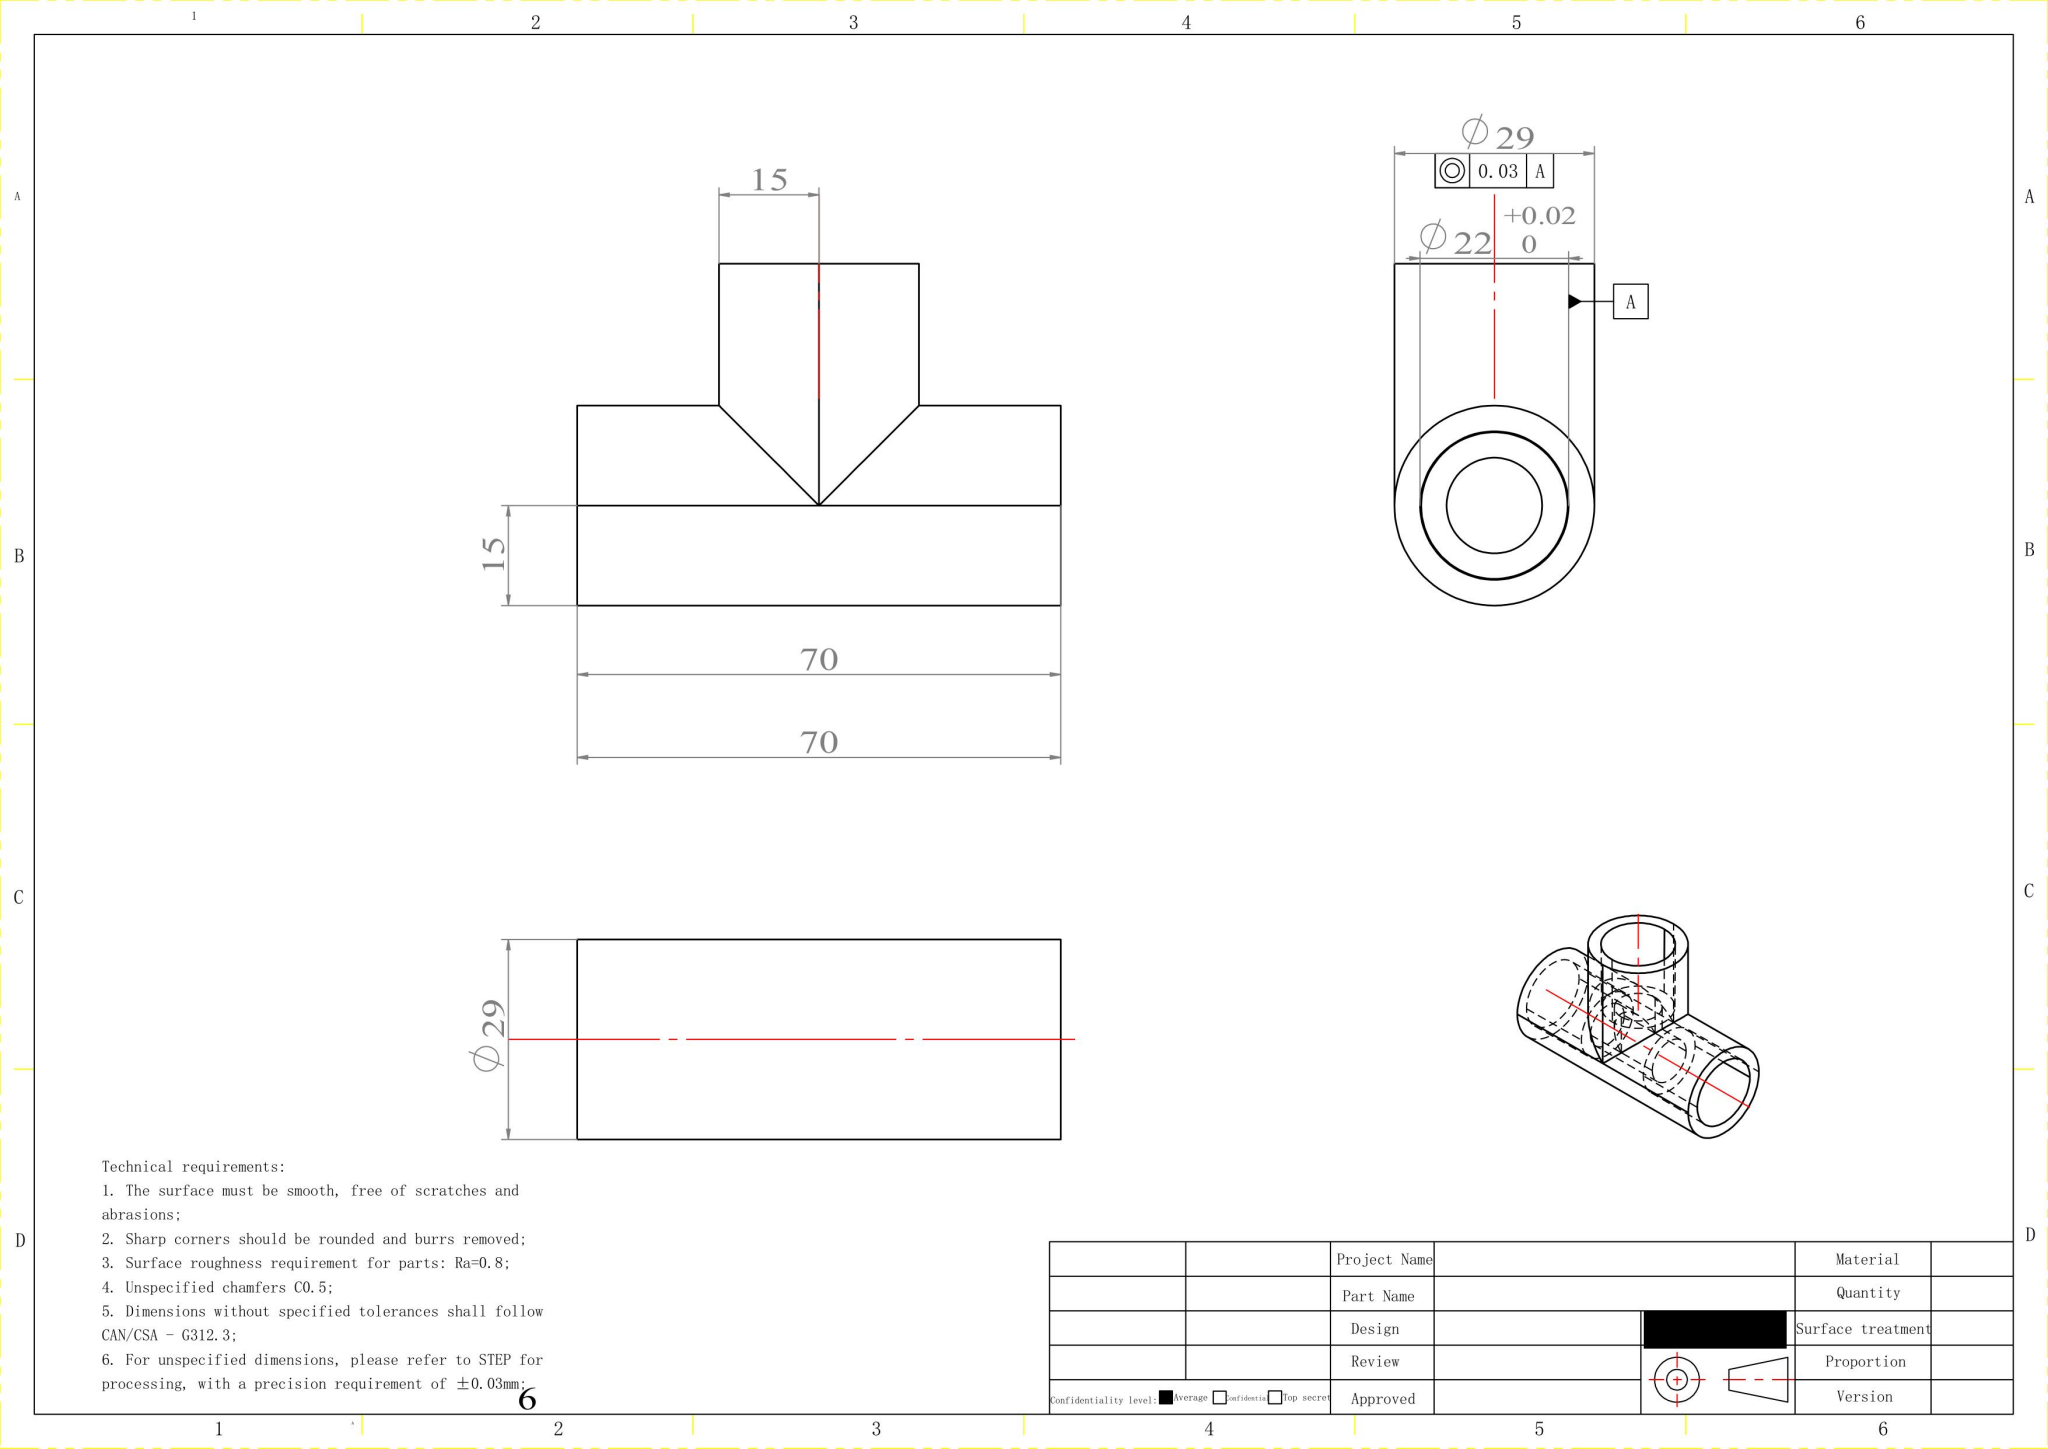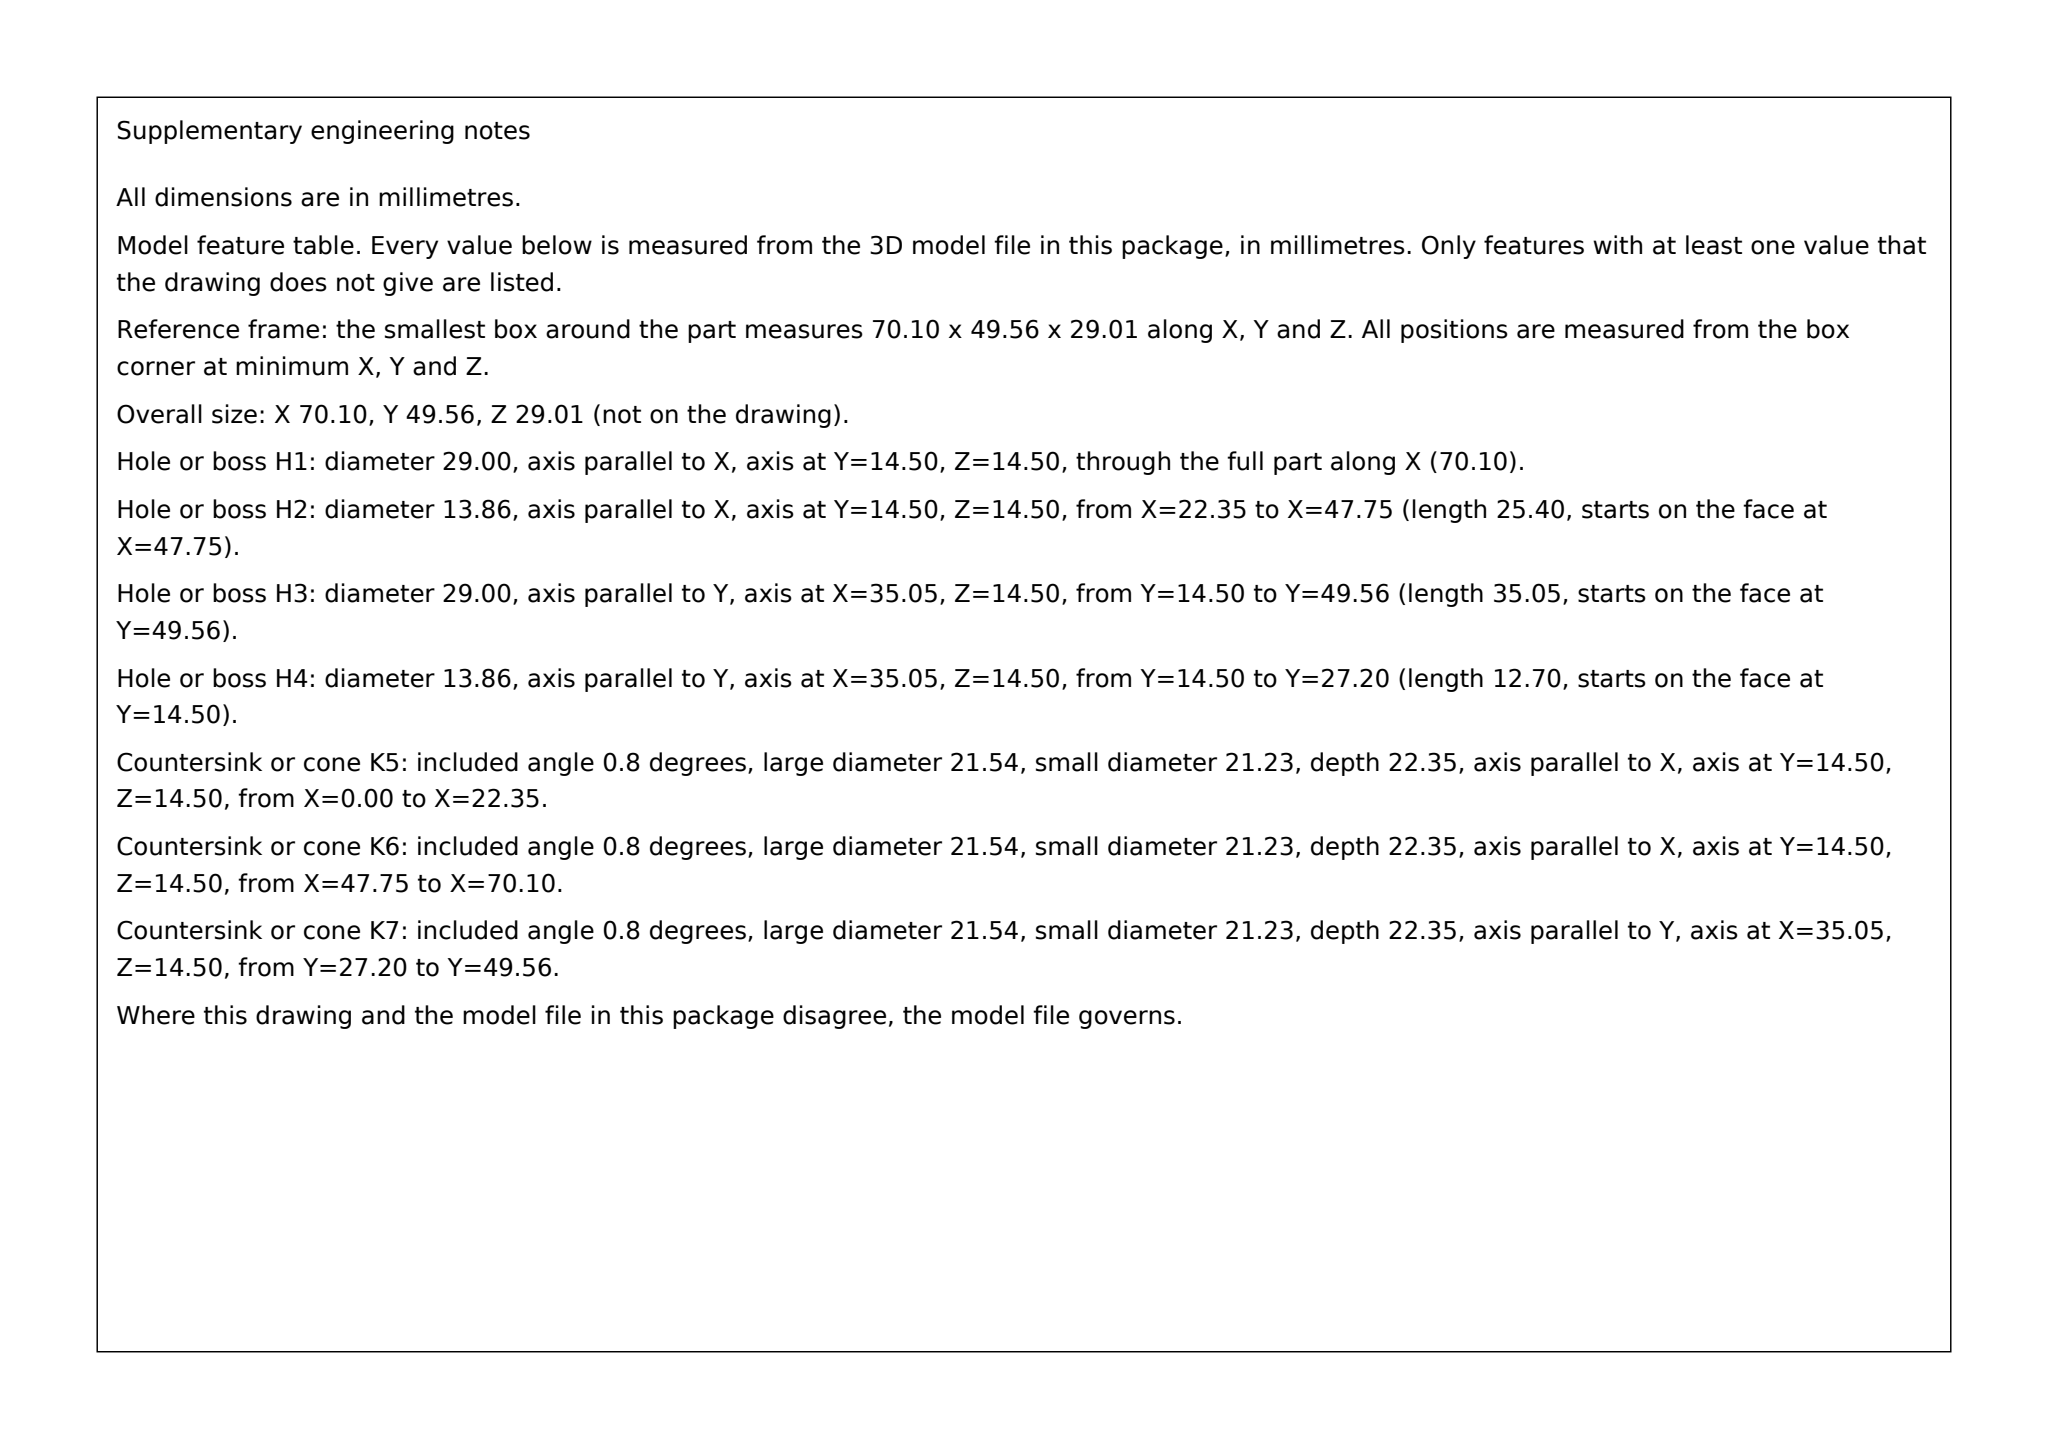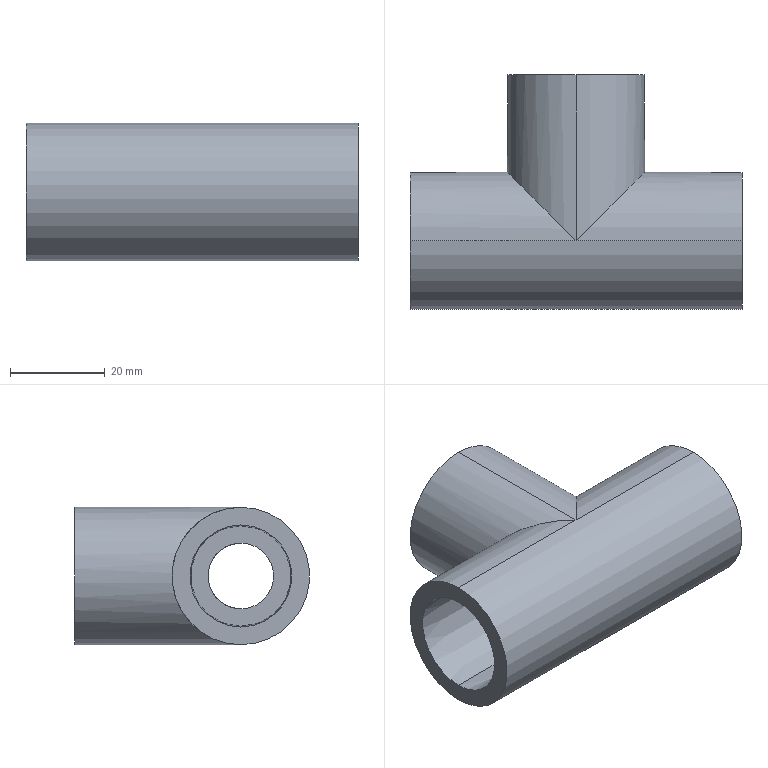Part | SolidWorks | mm | 1 solid | 22 faces | box 70.1 x 49.56 x 29.01 mm | volume 32399 mm3 | cylinder 10 | plane 6 | cone 6 | commonest cylinder face diameters 29.007 x5 13.868 x5
STEP:
#1=CARTESIAN_POINT('',(35.052,-0.,14.503));
#2=VERTEX_POINT('',#1);
#3=CARTESIAN_POINT('',(0.,0.,14.503));
#4=VERTEX_POINT('',#3);
#5=CARTESIAN_POINT('',(35.052,0.,14.503));
#6=DIRECTION('',(-1.,0.,0.));
#7=VECTOR('',#6,1000.);
#8=LINE('',#5,#7);
#9=EDGE_CURVE('',#2,#4,#8,.T.);
#10=ORIENTED_EDGE('',*,*,#9,.F.);
#11=CARTESIAN_POINT('',(35.052,-0.,-14.503));
#12=VERTEX_POINT('',#11);
#13=CARTESIAN_POINT('',(35.052,0.,-0.));
#14=DIRECTION('',(-1.,-0.,-0.));
#15=DIRECTION('',(0.,-0.,1.));
#16=AXIS2_PLACEMENT_3D('',#13,#14,#15);
#17=CIRCLE('',#16,14.503);
#18=EDGE_CURVE('',#2,#12,#17,.T.);
#19=ORIENTED_EDGE('',*,*,#18,.T.);
#20=CARTESIAN_POINT('',(0.,0.,-14.503));
#21=VERTEX_POINT('',#20);
#22=CARTESIAN_POINT('',(0.,0.,-14.503));
#23=DIRECTION('',(1.,-0.,0.));
#24=VECTOR('',#23,1000.);
#25=LINE('',#22,#24);
#26=EDGE_CURVE('',#21,#12,#25,.T.);
#27=ORIENTED_EDGE('',*,*,#26,.F.);
#28=CARTESIAN_POINT('',(0.,0.,14.503));
#29=CARTESIAN_POINT('',(14.503,14.503,14.503));
#30=CARTESIAN_POINT('',(14.503,14.503,0.));
#31=CARTESIAN_POINT('',(14.503,14.503,-14.503));
#32=CARTESIAN_POINT('',(0.,0.,-14.503));
#33=(BOUNDED_CURVE()B_SPLINE_CURVE(2,(#28,#29,#30,#31,#32),.UNSPECIFIED.,.F.,.F.)B_SPLINE_CURVE_WITH_KNOTS((3,2,3),(0.,0.5,1.),.UNSPECIFIED.)CURVE()GEOMETRIC_REPRESENTATION_ITEM()RATIONAL_B_SPLINE_CURVE((1.,0.7071,1.,0.7071,1.))REPRESENTATION_ITEM(''));
#34=EDGE_CURVE('',#4,#21,#33,.T.);
#35=ORIENTED_EDGE('',*,*,#34,.F.);
#36=EDGE_LOOP('',(#10,#19,#27,#35));
#37=FACE_OUTER_BOUND('',#36,.T.);
#38=CARTESIAN_POINT('',(35.052,0.,-0.));
#39=DIRECTION('',(-1.,0.,-0.));
#40=DIRECTION('',(-0.,0.,1.));
#41=AXIS2_PLACEMENT_3D('',#38,#39,#40);
#42=CYLINDRICAL_SURFACE('',#41,14.503);
#43=ADVANCED_FACE('',(#37),#42,.T.);
#44=CARTESIAN_POINT('',(-35.052,-0.,-14.503));
#45=VERTEX_POINT('',#44);
#46=CARTESIAN_POINT('',(-35.052,-0.,14.503));
#47=VERTEX_POINT('',#46);
#48=CARTESIAN_POINT('',(-35.052,-0.,-0.));
#49=DIRECTION('',(1.,0.,0.));
#50=DIRECTION('',(0.,0.,-1.));
#51=AXIS2_PLACEMENT_3D('',#48,#49,#50);
#52=CIRCLE('',#51,14.503);
#53=EDGE_CURVE('',#45,#47,#52,.T.);
#54=ORIENTED_EDGE('',*,*,#53,.T.);
#55=CARTESIAN_POINT('',(-35.052,0.,14.503));
#56=DIRECTION('',(1.,0.,0.));
#57=VECTOR('',#56,1000.);
#58=LINE('',#55,#57);
#59=EDGE_CURVE('',#47,#4,#58,.T.);
#60=ORIENTED_EDGE('',*,*,#59,.T.);
#61=CARTESIAN_POINT('',(0.,0.,-14.503));
#62=CARTESIAN_POINT('',(-14.503,14.503,-14.503));
#63=CARTESIAN_POINT('',(-14.503,14.503,-0.));
#64=CARTESIAN_POINT('',(-14.503,14.503,14.503));
#65=CARTESIAN_POINT('',(0.,0.,14.503));
#66=(BOUNDED_CURVE()B_SPLINE_CURVE(2,(#61,#62,#63,#64,#65),.UNSPECIFIED.,.F.,.F.)B_SPLINE_CURVE_WITH_KNOTS((3,2,3),(0.,0.5,1.),.UNSPECIFIED.)CURVE()GEOMETRIC_REPRESENTATION_ITEM()RATIONAL_B_SPLINE_CURVE((1.,0.7071,1.,0.7071,1.))REPRESENTATION_ITEM(''));
#67=EDGE_CURVE('',#21,#4,#66,.T.);
#68=ORIENTED_EDGE('',*,*,#67,.F.);
#69=CARTESIAN_POINT('',(-35.052,-0.,-14.503));
#70=DIRECTION('',(1.,0.,0.));
#71=VECTOR('',#70,1000.);
#72=LINE('',#69,#71);
#73=EDGE_CURVE('',#45,#21,#72,.T.);
#74=ORIENTED_EDGE('',*,*,#73,.F.);
#75=EDGE_LOOP('',(#54,#60,#68,#74));
#76=FACE_OUTER_BOUND('',#75,.T.);
#77=CARTESIAN_POINT('',(35.052,0.,-0.));
#78=DIRECTION('',(-1.,0.,-0.));
#79=DIRECTION('',(-0.,0.,1.));
#80=AXIS2_PLACEMENT_3D('',#77,#78,#79);
#81=CYLINDRICAL_SURFACE('',#80,14.503);
#82=ADVANCED_FACE('',(#76),#81,.T.);
#83=CARTESIAN_POINT('',(-12.7,0.,6.934));
#84=VERTEX_POINT('',#83);
#85=CARTESIAN_POINT('',(0.,0.,6.934));
#86=VERTEX_POINT('',#85);
#87=CARTESIAN_POINT('',(-12.7,0.,6.934));
#88=DIRECTION('',(1.,0.,0.));
#89=VECTOR('',#88,1000.);
#90=LINE('',#87,#89);
#91=EDGE_CURVE('',#84,#86,#90,.T.);
#92=ORIENTED_EDGE('',*,*,#91,.F.);
#93=CARTESIAN_POINT('',(-12.7,0.,-6.934));
#94=VERTEX_POINT('',#93);
#95=CARTESIAN_POINT('',(-12.7,0.,0.));
#96=DIRECTION('',(-1.,0.,0.));
#97=DIRECTION('',(0.,-0.,1.));
#98=AXIS2_PLACEMENT_3D('',#95,#96,#97);
#99=CIRCLE('',#98,6.934);
#100=EDGE_CURVE('',#84,#94,#99,.T.);
#101=ORIENTED_EDGE('',*,*,#100,.T.);
#102=CARTESIAN_POINT('',(0.,0.,-6.934));
#103=VERTEX_POINT('',#102);
#104=CARTESIAN_POINT('',(0.,0.,-6.934));
#105=DIRECTION('',(-1.,0.,0.));
#106=VECTOR('',#105,1000.);
#107=LINE('',#104,#106);
#108=EDGE_CURVE('',#103,#94,#107,.T.);
#109=ORIENTED_EDGE('',*,*,#108,.F.);
#110=CARTESIAN_POINT('',(0.,0.,6.934));
#111=CARTESIAN_POINT('',(-13.868,13.868,6.934));
#112=CARTESIAN_POINT('',(-13.868,13.868,-6.934));
#113=CARTESIAN_POINT('',(0.,0.,-6.934));
#114=(BOUNDED_CURVE()B_SPLINE_CURVE(3,(#110,#111,#112,#113),.UNSPECIFIED.,.F.,.F.)B_SPLINE_CURVE_WITH_KNOTS((4,4),(1.571,4.712),.UNSPECIFIED.)CURVE()GEOMETRIC_REPRESENTATION_ITEM()RATIONAL_B_SPLINE_CURVE((1.,0.3333,0.3333,1.))REPRESENTATION_ITEM(''));
#115=EDGE_CURVE('',#86,#103,#114,.T.);
#116=ORIENTED_EDGE('',*,*,#115,.F.);
#117=EDGE_LOOP('',(#92,#101,#109,#116));
#118=FACE_OUTER_BOUND('',#117,.T.);
#119=CARTESIAN_POINT('',(12.7,0.,0.));
#120=DIRECTION('',(-1.,0.,-0.));
#121=DIRECTION('',(-0.,-0.,1.));
#122=AXIS2_PLACEMENT_3D('',#119,#120,#121);
#123=CYLINDRICAL_SURFACE('',#122,6.934);
#124=ADVANCED_FACE('',(#118),#123,.F.);
#125=CARTESIAN_POINT('',(12.7,0.,-6.934));
#126=VERTEX_POINT('',#125);
#127=CARTESIAN_POINT('',(12.7,0.,6.934));
#128=VERTEX_POINT('',#127);
#129=CARTESIAN_POINT('',(12.7,0.,-0.));
#130=DIRECTION('',(1.,0.,-0.));
#131=DIRECTION('',(0.,-0.,-1.));
#132=AXIS2_PLACEMENT_3D('',#129,#130,#131);
#133=CIRCLE('',#132,6.934);
#134=EDGE_CURVE('',#126,#128,#133,.T.);
#135=ORIENTED_EDGE('',*,*,#134,.T.);
#136=CARTESIAN_POINT('',(12.7,0.,6.934));
#137=DIRECTION('',(-1.,0.,0.));
#138=VECTOR('',#137,1000.);
#139=LINE('',#136,#138);
#140=EDGE_CURVE('',#128,#86,#139,.T.);
#141=ORIENTED_EDGE('',*,*,#140,.T.);
#142=CARTESIAN_POINT('',(0.,0.,-6.934));
#143=CARTESIAN_POINT('',(13.868,13.868,-6.934));
#144=CARTESIAN_POINT('',(13.868,13.868,6.934));
#145=CARTESIAN_POINT('',(0.,0.,6.934));
#146=(BOUNDED_CURVE()B_SPLINE_CURVE(3,(#142,#143,#144,#145),.UNSPECIFIED.,.F.,.T.)B_SPLINE_CURVE_WITH_KNOTS((4,4),(1.571,4.712),.UNSPECIFIED.)CURVE()GEOMETRIC_REPRESENTATION_ITEM()RATIONAL_B_SPLINE_CURVE((1.,0.3333,0.3333,1.))REPRESENTATION_ITEM(''));
#147=EDGE_CURVE('',#103,#86,#146,.T.);
#148=ORIENTED_EDGE('',*,*,#147,.F.);
#149=CARTESIAN_POINT('',(12.7,0.,-6.934));
#150=DIRECTION('',(-1.,-0.,0.));
#151=VECTOR('',#150,1000.);
#152=LINE('',#149,#151);
#153=EDGE_CURVE('',#126,#103,#152,.T.);
#154=ORIENTED_EDGE('',*,*,#153,.F.);
#155=EDGE_LOOP('',(#135,#141,#148,#154));
#156=FACE_OUTER_BOUND('',#155,.T.);
#157=CARTESIAN_POINT('',(12.7,0.,0.));
#158=DIRECTION('',(-1.,0.,-0.));
#159=DIRECTION('',(-0.,-0.,1.));
#160=AXIS2_PLACEMENT_3D('',#157,#158,#159);
#161=CYLINDRICAL_SURFACE('',#160,6.934);
#162=ADVANCED_FACE('',(#156),#161,.F.);
#163=CARTESIAN_POINT('',(12.7,0.,0.));
#164=DIRECTION('',(1.,0.,0.));
#165=DIRECTION('',(-0.,0.,1.));
#166=AXIS2_PLACEMENT_3D('',#163,#164,#165);
#167=CIRCLE('',#166,6.934);
#168=EDGE_CURVE('',#128,#126,#167,.T.);
#169=ORIENTED_EDGE('',*,*,#168,.F.);
#170=ORIENTED_EDGE('',*,*,#134,.F.);
#171=EDGE_LOOP('',(#169,#170));
#172=FACE_BOUND('',#171,.T.);
#173=CARTESIAN_POINT('',(12.7,0.,10.617));
#174=VERTEX_POINT('',#173);
#175=CARTESIAN_POINT('',(12.7,0.,-10.617));
#176=VERTEX_POINT('',#175);
#177=CARTESIAN_POINT('',(12.7,0.,0.));
#178=DIRECTION('',(-1.,0.,0.));
#179=DIRECTION('',(0.,-0.,1.));
#180=AXIS2_PLACEMENT_3D('',#177,#178,#179);
#181=CIRCLE('',#180,10.617);
#182=EDGE_CURVE('',#174,#176,#181,.T.);
#183=ORIENTED_EDGE('',*,*,#182,.F.);
#184=CARTESIAN_POINT('',(12.7,-0.,-0.));
#185=DIRECTION('',(-1.,0.,0.));
#186=DIRECTION('',(0.,0.,-1.));
#187=AXIS2_PLACEMENT_3D('',#184,#185,#186);
#188=CIRCLE('',#187,10.617);
#189=EDGE_CURVE('',#176,#174,#188,.T.);
#190=ORIENTED_EDGE('',*,*,#189,.F.);
#191=EDGE_LOOP('',(#183,#190));
#192=FACE_OUTER_BOUND('',#191,.T.);
#193=CARTESIAN_POINT('',(12.7,-14.503,0.));
#194=DIRECTION('',(1.,0.,0.));
#195=DIRECTION('',(0.,1.,0.));
#196=AXIS2_PLACEMENT_3D('',#193,#194,#195);
#197=PLANE('',#196);
#198=ADVANCED_FACE('',(#172,#192),#197,.T.);
#199=CARTESIAN_POINT('',(35.052,0.,10.77));
#200=VERTEX_POINT('',#199);
#201=CARTESIAN_POINT('',(35.052,0.,-10.77));
#202=VERTEX_POINT('',#201);
#203=CARTESIAN_POINT('',(35.052,-0.,-0.));
#204=DIRECTION('',(1.,-0.,-0.));
#205=DIRECTION('',(0.,-0.,1.));
#206=AXIS2_PLACEMENT_3D('',#203,#204,#205);
#207=CIRCLE('',#206,10.77);
#208=EDGE_CURVE('',#200,#202,#207,.T.);
#209=ORIENTED_EDGE('',*,*,#208,.F.);
#210=CARTESIAN_POINT('',(35.052,0.,-0.));
#211=DIRECTION('',(1.,-0.,-0.));
#212=DIRECTION('',(0.,0.,-1.));
#213=AXIS2_PLACEMENT_3D('',#210,#211,#212);
#214=CIRCLE('',#213,10.77);
#215=EDGE_CURVE('',#202,#200,#214,.T.);
#216=ORIENTED_EDGE('',*,*,#215,.F.);
#217=EDGE_LOOP('',(#209,#216));
#218=FACE_BOUND('',#217,.T.);
#219=ORIENTED_EDGE('',*,*,#18,.F.);
#220=CARTESIAN_POINT('',(35.052,0.,0.));
#221=DIRECTION('',(-1.,-0.,0.));
#222=DIRECTION('',(0.,-0.,-1.));
#223=AXIS2_PLACEMENT_3D('',#220,#221,#222);
#224=CIRCLE('',#223,14.503);
#225=EDGE_CURVE('',#12,#2,#224,.T.);
#226=ORIENTED_EDGE('',*,*,#225,.F.);
#227=EDGE_LOOP('',(#219,#226));
#228=FACE_OUTER_BOUND('',#227,.T.);
#229=CARTESIAN_POINT('',(35.052,-14.503,0.));
#230=DIRECTION('',(1.,0.,0.));
#231=DIRECTION('',(0.,1.,0.));
#232=AXIS2_PLACEMENT_3D('',#229,#230,#231);
#233=PLANE('',#232);
#234=ADVANCED_FACE('',(#218,#228),#233,.T.);
#235=CARTESIAN_POINT('',(0.,35.052,10.77));
#236=VERTEX_POINT('',#235);
#237=CARTESIAN_POINT('',(-0.,35.052,-10.77));
#238=VERTEX_POINT('',#237);
#239=CARTESIAN_POINT('',(0.,35.052,0.));
#240=DIRECTION('',(-0.,1.,0.));
#241=DIRECTION('',(0.,0.,1.));
#242=AXIS2_PLACEMENT_3D('',#239,#240,#241);
#243=CIRCLE('',#242,10.77);
#244=EDGE_CURVE('',#236,#238,#243,.T.);
#245=ORIENTED_EDGE('',*,*,#244,.F.);
#246=CARTESIAN_POINT('',(0.,35.052,-0.));
#247=DIRECTION('',(0.,1.,-0.));
#248=DIRECTION('',(-0.,0.,-1.));
#249=AXIS2_PLACEMENT_3D('',#246,#247,#248);
#250=CIRCLE('',#249,10.77);
#251=EDGE_CURVE('',#238,#236,#250,.T.);
#252=ORIENTED_EDGE('',*,*,#251,.F.);
#253=EDGE_LOOP('',(#245,#252));
#254=FACE_BOUND('',#253,.T.);
#255=CARTESIAN_POINT('',(-0.,35.052,-14.503));
#256=VERTEX_POINT('',#255);
#257=CARTESIAN_POINT('',(-0.,35.052,14.503));
#258=VERTEX_POINT('',#257);
#259=CARTESIAN_POINT('',(0.,35.052,0.));
#260=DIRECTION('',(-0.,-1.,0.));
#261=DIRECTION('',(-0.,0.,-1.));
#262=AXIS2_PLACEMENT_3D('',#259,#260,#261);
#263=CIRCLE('',#262,14.503);
#264=EDGE_CURVE('',#256,#258,#263,.T.);
#265=ORIENTED_EDGE('',*,*,#264,.F.);
#266=CARTESIAN_POINT('',(0.,35.052,-0.));
#267=DIRECTION('',(-0.,-1.,-0.));
#268=DIRECTION('',(-0.,0.,1.));
#269=AXIS2_PLACEMENT_3D('',#266,#267,#268);
#270=CIRCLE('',#269,14.503);
#271=EDGE_CURVE('',#258,#256,#270,.T.);
#272=ORIENTED_EDGE('',*,*,#271,.F.);
#273=EDGE_LOOP('',(#265,#272));
#274=FACE_OUTER_BOUND('',#273,.T.);
#275=CARTESIAN_POINT('',(14.503,35.052,0.));
#276=DIRECTION('',(0.,1.,0.));
#277=DIRECTION('',(1.,0.,0.));
#278=AXIS2_PLACEMENT_3D('',#275,#276,#277);
#279=PLANE('',#278);
#280=ADVANCED_FACE('',(#254,#274),#279,.T.);
#281=ORIENTED_EDGE('',*,*,#100,.F.);
#282=CARTESIAN_POINT('',(-12.7,0.,-0.));
#283=DIRECTION('',(-1.,0.,0.));
#284=DIRECTION('',(0.,0.,-1.));
#285=AXIS2_PLACEMENT_3D('',#282,#283,#284);
#286=CIRCLE('',#285,6.934);
#287=EDGE_CURVE('',#94,#84,#286,.T.);
#288=ORIENTED_EDGE('',*,*,#287,.F.);
#289=EDGE_LOOP('',(#281,#288));
#290=FACE_BOUND('',#289,.T.);
#291=CARTESIAN_POINT('',(-12.7,0.,10.617));
#292=VERTEX_POINT('',#291);
#293=CARTESIAN_POINT('',(-12.7,-0.,-10.617));
#294=VERTEX_POINT('',#293);
#295=CARTESIAN_POINT('',(-12.7,-0.,0.));
#296=DIRECTION('',(1.,0.,0.));
#297=DIRECTION('',(0.,0.,1.));
#298=AXIS2_PLACEMENT_3D('',#295,#296,#297);
#299=CIRCLE('',#298,10.617);
#300=EDGE_CURVE('',#292,#294,#299,.T.);
#301=ORIENTED_EDGE('',*,*,#300,.F.);
#302=CARTESIAN_POINT('',(-12.7,0.,-0.));
#303=DIRECTION('',(1.,0.,0.));
#304=DIRECTION('',(0.,-0.,-1.));
#305=AXIS2_PLACEMENT_3D('',#302,#303,#304);
#306=CIRCLE('',#305,10.617);
#307=EDGE_CURVE('',#294,#292,#306,.T.);
#308=ORIENTED_EDGE('',*,*,#307,.F.);
#309=EDGE_LOOP('',(#301,#308));
#310=FACE_OUTER_BOUND('',#309,.T.);
#311=CARTESIAN_POINT('',(-12.7,0.,0.));
#312=DIRECTION('',(-1.,0.,0.));
#313=DIRECTION('',(0.,0.,1.));
#314=AXIS2_PLACEMENT_3D('',#311,#312,#313);
#315=PLANE('',#314);
#316=ADVANCED_FACE('',(#290,#310),#315,.T.);
#317=CARTESIAN_POINT('',(0.,12.7,6.934));
#318=VERTEX_POINT('',#317);
#319=CARTESIAN_POINT('',(-0.,12.7,-6.934));
#320=VERTEX_POINT('',#319);
#321=CARTESIAN_POINT('',(-0.,12.7,0.));
#322=DIRECTION('',(0.,1.,0.));
#323=DIRECTION('',(0.,-0.,1.));
#324=AXIS2_PLACEMENT_3D('',#321,#322,#323);
#325=CIRCLE('',#324,6.934);
#326=EDGE_CURVE('',#318,#320,#325,.T.);
#327=ORIENTED_EDGE('',*,*,#326,.F.);
#328=CARTESIAN_POINT('',(-0.,12.7,-0.));
#329=DIRECTION('',(0.,1.,0.));
#330=DIRECTION('',(0.,0.,-1.));
#331=AXIS2_PLACEMENT_3D('',#328,#329,#330);
#332=CIRCLE('',#331,6.934);
#333=EDGE_CURVE('',#320,#318,#332,.T.);
#334=ORIENTED_EDGE('',*,*,#333,.F.);
#335=EDGE_LOOP('',(#327,#334));
#336=FACE_BOUND('',#335,.T.);
#337=CARTESIAN_POINT('',(0.,12.7,10.617));
#338=VERTEX_POINT('',#337);
#339=CARTESIAN_POINT('',(-0.,12.7,-10.617));
#340=VERTEX_POINT('',#339);
#341=CARTESIAN_POINT('',(-0.,12.7,0.));
#342=DIRECTION('',(0.,-1.,0.));
#343=DIRECTION('',(0.,0.,1.));
#344=AXIS2_PLACEMENT_3D('',#341,#342,#343);
#345=CIRCLE('',#344,10.617);
#346=EDGE_CURVE('',#338,#340,#345,.T.);
#347=ORIENTED_EDGE('',*,*,#346,.F.);
#348=CARTESIAN_POINT('',(0.,12.7,-0.));
#349=DIRECTION('',(0.,-1.,0.));
#350=DIRECTION('',(-0.,0.,-1.));
#351=AXIS2_PLACEMENT_3D('',#348,#349,#350);
#352=CIRCLE('',#351,10.617);
#353=EDGE_CURVE('',#340,#338,#352,.T.);
#354=ORIENTED_EDGE('',*,*,#353,.F.);
#355=EDGE_LOOP('',(#347,#354));
#356=FACE_OUTER_BOUND('',#355,.T.);
#357=CARTESIAN_POINT('',(52.467,12.7,-7.004));
#358=DIRECTION('',(0.,1.,0.));
#359=DIRECTION('',(1.,0.,0.));
#360=AXIS2_PLACEMENT_3D('',#357,#358,#359);
#361=PLANE('',#360);
#362=ADVANCED_FACE('',(#336,#356),#361,.T.);
#363=CARTESIAN_POINT('',(-35.052,-0.,10.77));
#364=VERTEX_POINT('',#363);
#365=CARTESIAN_POINT('',(-35.052,-0.,-10.77));
#366=VERTEX_POINT('',#365);
#367=CARTESIAN_POINT('',(-35.052,-0.,0.));
#368=DIRECTION('',(-1.,-0.,0.));
#369=DIRECTION('',(0.,0.,1.));
#370=AXIS2_PLACEMENT_3D('',#367,#368,#369);
#371=CIRCLE('',#370,10.77);
#372=EDGE_CURVE('',#364,#366,#371,.T.);
#373=ORIENTED_EDGE('',*,*,#372,.F.);
#374=CARTESIAN_POINT('',(-35.052,0.,0.));
#375=DIRECTION('',(-1.,0.,-0.));
#376=DIRECTION('',(0.,-0.,-1.));
#377=AXIS2_PLACEMENT_3D('',#374,#375,#376);
#378=CIRCLE('',#377,10.77);
#379=EDGE_CURVE('',#366,#364,#378,.T.);
#380=ORIENTED_EDGE('',*,*,#379,.F.);
#381=EDGE_LOOP('',(#373,#380));
#382=FACE_BOUND('',#381,.T.);
#383=CARTESIAN_POINT('',(-35.052,-0.,-0.));
#384=DIRECTION('',(1.,0.,-0.));
#385=DIRECTION('',(0.,0.,1.));
#386=AXIS2_PLACEMENT_3D('',#383,#384,#385);
#387=CIRCLE('',#386,14.503);
#388=EDGE_CURVE('',#47,#45,#387,.T.);
#389=ORIENTED_EDGE('',*,*,#388,.F.);
#390=ORIENTED_EDGE('',*,*,#53,.F.);
#391=EDGE_LOOP('',(#389,#390));
#392=FACE_OUTER_BOUND('',#391,.T.);
#393=CARTESIAN_POINT('',(-35.052,-14.503,0.));
#394=DIRECTION('',(-1.,0.,0.));
#395=DIRECTION('',(0.,0.,1.));
#396=AXIS2_PLACEMENT_3D('',#393,#394,#395);
#397=PLANE('',#396);
#398=ADVANCED_FACE('',(#382,#392),#397,.T.);
#399=ORIENTED_EDGE('',*,*,#73,.T.);
#400=ORIENTED_EDGE('',*,*,#26,.T.);
#401=ORIENTED_EDGE('',*,*,#225,.T.);
#402=ORIENTED_EDGE('',*,*,#9,.T.);
#403=ORIENTED_EDGE('',*,*,#59,.F.);
#404=ORIENTED_EDGE('',*,*,#388,.T.);
#405=EDGE_LOOP('',(#399,#400,#401,#402,#403,#404));
#406=FACE_OUTER_BOUND('',#405,.T.);
#407=CARTESIAN_POINT('',(35.052,0.,-0.));
#408=DIRECTION('',(-1.,0.,-0.));
#409=DIRECTION('',(-0.,0.,1.));
#410=AXIS2_PLACEMENT_3D('',#407,#408,#409);
#411=CYLINDRICAL_SURFACE('',#410,14.503);
#412=ADVANCED_FACE('',(#406),#411,.T.);
#413=ORIENTED_EDGE('',*,*,#307,.T.);
#414=CARTESIAN_POINT('',(-35.052,0.,10.77));
#415=DIRECTION('',(1.,0.,-0.006818));
#416=VECTOR('',#415,1000.);
#417=LINE('',#414,#416);
#418=EDGE_CURVE('',#364,#292,#417,.T.);
#419=ORIENTED_EDGE('',*,*,#418,.F.);
#420=ORIENTED_EDGE('',*,*,#372,.T.);
#421=CARTESIAN_POINT('',(-12.7,-0.,-10.617));
#422=DIRECTION('',(-1.,-0.,-0.006818));
#423=VECTOR('',#422,1000.);
#424=LINE('',#421,#423);
#425=EDGE_CURVE('',#294,#366,#424,.T.);
#426=ORIENTED_EDGE('',*,*,#425,.F.);
#427=EDGE_LOOP('',(#413,#419,#420,#426));
#428=FACE_OUTER_BOUND('',#427,.T.);
#429=CARTESIAN_POINT('',(36.258,0.,0.));
#430=DIRECTION('',(-1.,0.,0.));
#431=DIRECTION('',(0.,-0.,1.));
#432=AXIS2_PLACEMENT_3D('',#429,#430,#431);
#433=CONICAL_SURFACE('',#432,10.283,0.006818);
#434=ADVANCED_FACE('',(#428),#433,.F.);
#435=ORIENTED_EDGE('',*,*,#425,.T.);
#436=ORIENTED_EDGE('',*,*,#379,.T.);
#437=ORIENTED_EDGE('',*,*,#418,.T.);
#438=ORIENTED_EDGE('',*,*,#300,.T.);
#439=EDGE_LOOP('',(#435,#436,#437,#438));
#440=FACE_OUTER_BOUND('',#439,.T.);
#441=CARTESIAN_POINT('',(36.258,0.,0.));
#442=DIRECTION('',(-1.,0.,0.));
#443=DIRECTION('',(0.,-0.,1.));
#444=AXIS2_PLACEMENT_3D('',#441,#442,#443);
#445=CONICAL_SURFACE('',#444,10.283,0.006818);
#446=ADVANCED_FACE('',(#440),#445,.F.);
#447=ORIENTED_EDGE('',*,*,#67,.T.);
#448=CARTESIAN_POINT('',(0.,0.,14.503));
#449=DIRECTION('',(-0.,1.,0.));
#450=VECTOR('',#449,1000.);
#451=LINE('',#448,#450);
#452=EDGE_CURVE('',#4,#258,#451,.T.);
#453=ORIENTED_EDGE('',*,*,#452,.T.);
#454=ORIENTED_EDGE('',*,*,#271,.T.);
#455=CARTESIAN_POINT('',(0.,-0.,-14.503));
#456=DIRECTION('',(0.,1.,0.));
#457=VECTOR('',#456,1000.);
#458=LINE('',#455,#457);
#459=EDGE_CURVE('',#21,#256,#458,.T.);
#460=ORIENTED_EDGE('',*,*,#459,.F.);
#461=EDGE_LOOP('',(#447,#453,#454,#460));
#462=FACE_OUTER_BOUND('',#461,.T.);
#463=CARTESIAN_POINT('',(-0.,35.052,-0.));
#464=DIRECTION('',(0.,-1.,0.));
#465=DIRECTION('',(0.,0.,-1.));
#466=AXIS2_PLACEMENT_3D('',#463,#464,#465);
#467=CYLINDRICAL_SURFACE('',#466,14.503);
#468=ADVANCED_FACE('',(#462),#467,.T.);
#469=ORIENTED_EDGE('',*,*,#452,.F.);
#470=ORIENTED_EDGE('',*,*,#34,.T.);
#471=ORIENTED_EDGE('',*,*,#459,.T.);
#472=ORIENTED_EDGE('',*,*,#264,.T.);
#473=EDGE_LOOP('',(#469,#470,#471,#472));
#474=FACE_OUTER_BOUND('',#473,.T.);
#475=CARTESIAN_POINT('',(-0.,35.052,-0.));
#476=DIRECTION('',(0.,-1.,0.));
#477=DIRECTION('',(0.,0.,-1.));
#478=AXIS2_PLACEMENT_3D('',#475,#476,#477);
#479=CYLINDRICAL_SURFACE('',#478,14.503);
#480=ADVANCED_FACE('',(#474),#479,.T.);
#481=ORIENTED_EDGE('',*,*,#353,.T.);
#482=CARTESIAN_POINT('',(0.,35.052,10.77));
#483=DIRECTION('',(0.,-1.,-0.006818));
#484=VECTOR('',#483,1000.);
#485=LINE('',#482,#484);
#486=EDGE_CURVE('',#236,#338,#485,.T.);
#487=ORIENTED_EDGE('',*,*,#486,.F.);
#488=ORIENTED_EDGE('',*,*,#244,.T.);
#489=CARTESIAN_POINT('',(-0.,12.7,-10.617));
#490=DIRECTION('',(-0.,1.,-0.006818));
#491=VECTOR('',#490,1000.);
#492=LINE('',#489,#491);
#493=EDGE_CURVE('',#340,#238,#492,.T.);
#494=ORIENTED_EDGE('',*,*,#493,.F.);
#495=EDGE_LOOP('',(#481,#487,#488,#494));
#496=FACE_OUTER_BOUND('',#495,.T.);
#497=CARTESIAN_POINT('',(-0.,-13.906,-0.));
#498=DIRECTION('',(0.,1.,0.));
#499=DIRECTION('',(0.,0.,1.));
#500=AXIS2_PLACEMENT_3D('',#497,#498,#499);
#501=CONICAL_SURFACE('',#500,10.436,0.006818);
#502=ADVANCED_FACE('',(#496),#501,.F.);
#503=ORIENTED_EDGE('',*,*,#493,.T.);
#504=ORIENTED_EDGE('',*,*,#251,.T.);
#505=ORIENTED_EDGE('',*,*,#486,.T.);
#506=ORIENTED_EDGE('',*,*,#346,.T.);
#507=EDGE_LOOP('',(#503,#504,#505,#506));
#508=FACE_OUTER_BOUND('',#507,.T.);
#509=CARTESIAN_POINT('',(-0.,-13.906,-0.));
#510=DIRECTION('',(0.,1.,0.));
#511=DIRECTION('',(0.,0.,1.));
#512=AXIS2_PLACEMENT_3D('',#509,#510,#511);
#513=CONICAL_SURFACE('',#512,10.436,0.006818);
#514=ADVANCED_FACE('',(#508),#513,.F.);
#515=ORIENTED_EDGE('',*,*,#189,.T.);
#516=CARTESIAN_POINT('',(35.052,0.,10.77));
#517=DIRECTION('',(-1.,0.,-0.006818));
#518=VECTOR('',#517,1000.);
#519=LINE('',#516,#518);
#520=EDGE_CURVE('',#200,#174,#519,.T.);
#521=ORIENTED_EDGE('',*,*,#520,.F.);
#522=ORIENTED_EDGE('',*,*,#208,.T.);
#523=CARTESIAN_POINT('',(12.7,0.,-10.617));
#524=DIRECTION('',(1.,0.,-0.006818));
#525=VECTOR('',#524,1000.);
#526=LINE('',#523,#525);
#527=EDGE_CURVE('',#176,#202,#526,.T.);
#528=ORIENTED_EDGE('',*,*,#527,.F.);
#529=EDGE_LOOP('',(#515,#521,#522,#528));
#530=FACE_OUTER_BOUND('',#529,.T.);
#531=CARTESIAN_POINT('',(-36.258,-0.,0.));
#532=DIRECTION('',(1.,-0.,0.));
#533=DIRECTION('',(-0.,0.,1.));
#534=AXIS2_PLACEMENT_3D('',#531,#532,#533);
#535=CONICAL_SURFACE('',#534,10.283,0.006818);
#536=ADVANCED_FACE('',(#530),#535,.F.);
#537=ORIENTED_EDGE('',*,*,#527,.T.);
#538=ORIENTED_EDGE('',*,*,#215,.T.);
#539=ORIENTED_EDGE('',*,*,#520,.T.);
#540=ORIENTED_EDGE('',*,*,#182,.T.);
#541=EDGE_LOOP('',(#537,#538,#539,#540));
#542=FACE_OUTER_BOUND('',#541,.T.);
#543=CARTESIAN_POINT('',(-36.258,-0.,0.));
#544=DIRECTION('',(1.,-0.,0.));
#545=DIRECTION('',(-0.,0.,1.));
#546=AXIS2_PLACEMENT_3D('',#543,#544,#545);
#547=CONICAL_SURFACE('',#546,10.283,0.006818);
#548=ADVANCED_FACE('',(#542),#547,.F.);
#549=ORIENTED_EDGE('',*,*,#153,.T.);
#550=ORIENTED_EDGE('',*,*,#108,.T.);
#551=ORIENTED_EDGE('',*,*,#287,.T.);
#552=ORIENTED_EDGE('',*,*,#91,.T.);
#553=ORIENTED_EDGE('',*,*,#140,.F.);
#554=ORIENTED_EDGE('',*,*,#168,.T.);
#555=EDGE_LOOP('',(#549,#550,#551,#552,#553,#554));
#556=FACE_OUTER_BOUND('',#555,.T.);
#557=CARTESIAN_POINT('',(12.7,0.,0.));
#558=DIRECTION('',(-1.,0.,-0.));
#559=DIRECTION('',(-0.,-0.,1.));
#560=AXIS2_PLACEMENT_3D('',#557,#558,#559);
#561=CYLINDRICAL_SURFACE('',#560,6.934);
#562=ADVANCED_FACE('',(#556),#561,.F.);
#563=ORIENTED_EDGE('',*,*,#115,.T.);
#564=CARTESIAN_POINT('',(0.,0.,-6.934));
#565=DIRECTION('',(-0.,1.,0.));
#566=VECTOR('',#565,1000.);
#567=LINE('',#564,#566);
#568=EDGE_CURVE('',#103,#320,#567,.T.);
#569=ORIENTED_EDGE('',*,*,#568,.T.);
#570=ORIENTED_EDGE('',*,*,#333,.T.);
#571=CARTESIAN_POINT('',(0.,-0.,6.934));
#572=DIRECTION('',(0.,1.,0.));
#573=VECTOR('',#572,1000.);
#574=LINE('',#571,#573);
#575=EDGE_CURVE('',#86,#318,#574,.T.);
#576=ORIENTED_EDGE('',*,*,#575,.F.);
#577=EDGE_LOOP('',(#563,#569,#570,#576));
#578=FACE_OUTER_BOUND('',#577,.T.);
#579=CARTESIAN_POINT('',(0.,-0.,0.));
#580=DIRECTION('',(0.,1.,-0.));
#581=DIRECTION('',(-0.,0.,1.));
#582=AXIS2_PLACEMENT_3D('',#579,#580,#581);
#583=CYLINDRICAL_SURFACE('',#582,6.934);
#584=ADVANCED_FACE('',(#578),#583,.F.);
#585=ORIENTED_EDGE('',*,*,#568,.F.);
#586=ORIENTED_EDGE('',*,*,#147,.T.);
#587=ORIENTED_EDGE('',*,*,#575,.T.);
#588=ORIENTED_EDGE('',*,*,#326,.T.);
#589=EDGE_LOOP('',(#585,#586,#587,#588));
#590=FACE_OUTER_BOUND('',#589,.T.);
#591=CARTESIAN_POINT('',(0.,-0.,0.));
#592=DIRECTION('',(0.,1.,-0.));
#593=DIRECTION('',(-0.,0.,1.));
#594=AXIS2_PLACEMENT_3D('',#591,#592,#593);
#595=CYLINDRICAL_SURFACE('',#594,6.934);
#596=ADVANCED_FACE('',(#590),#595,.F.);
#597=CLOSED_SHELL('',(#43,#82,#124,#162,#198,#234,#280,#316,#362,#398,#412,#434,#446,#468,#480,#502,#514,#536,#548,#562,#584,#596));
#598=MANIFOLD_SOLID_BREP('',#597);
#599=CARTESIAN_POINT('',(0.,0.,0.));
#600=DIRECTION('',(0.,0.,1.));
#601=DIRECTION('',(1.,0.,0.));
#602=AXIS2_PLACEMENT_3D('',#599,#600,#601);
#603=(LENGTH_UNIT()NAMED_UNIT(*)SI_UNIT(.MILLI.,.METRE.));
#604=UNCERTAINTY_MEASURE_WITH_UNIT(LENGTH_MEASURE(0.00001),#603,'','');
#605=(NAMED_UNIT(*)PLANE_ANGLE_UNIT()SI_UNIT($,.RADIAN.));
#606=(NAMED_UNIT(*)SI_UNIT($,.STERADIAN.)SOLID_ANGLE_UNIT());
#607=(GEOMETRIC_REPRESENTATION_CONTEXT(3)GLOBAL_UNCERTAINTY_ASSIGNED_CONTEXT((#604))GLOBAL_UNIT_ASSIGNED_CONTEXT((#603,#605,#606))REPRESENTATION_CONTEXT('',''));
#608=ADVANCED_BREP_SHAPE_REPRESENTATION('',(#598,#602),#607);